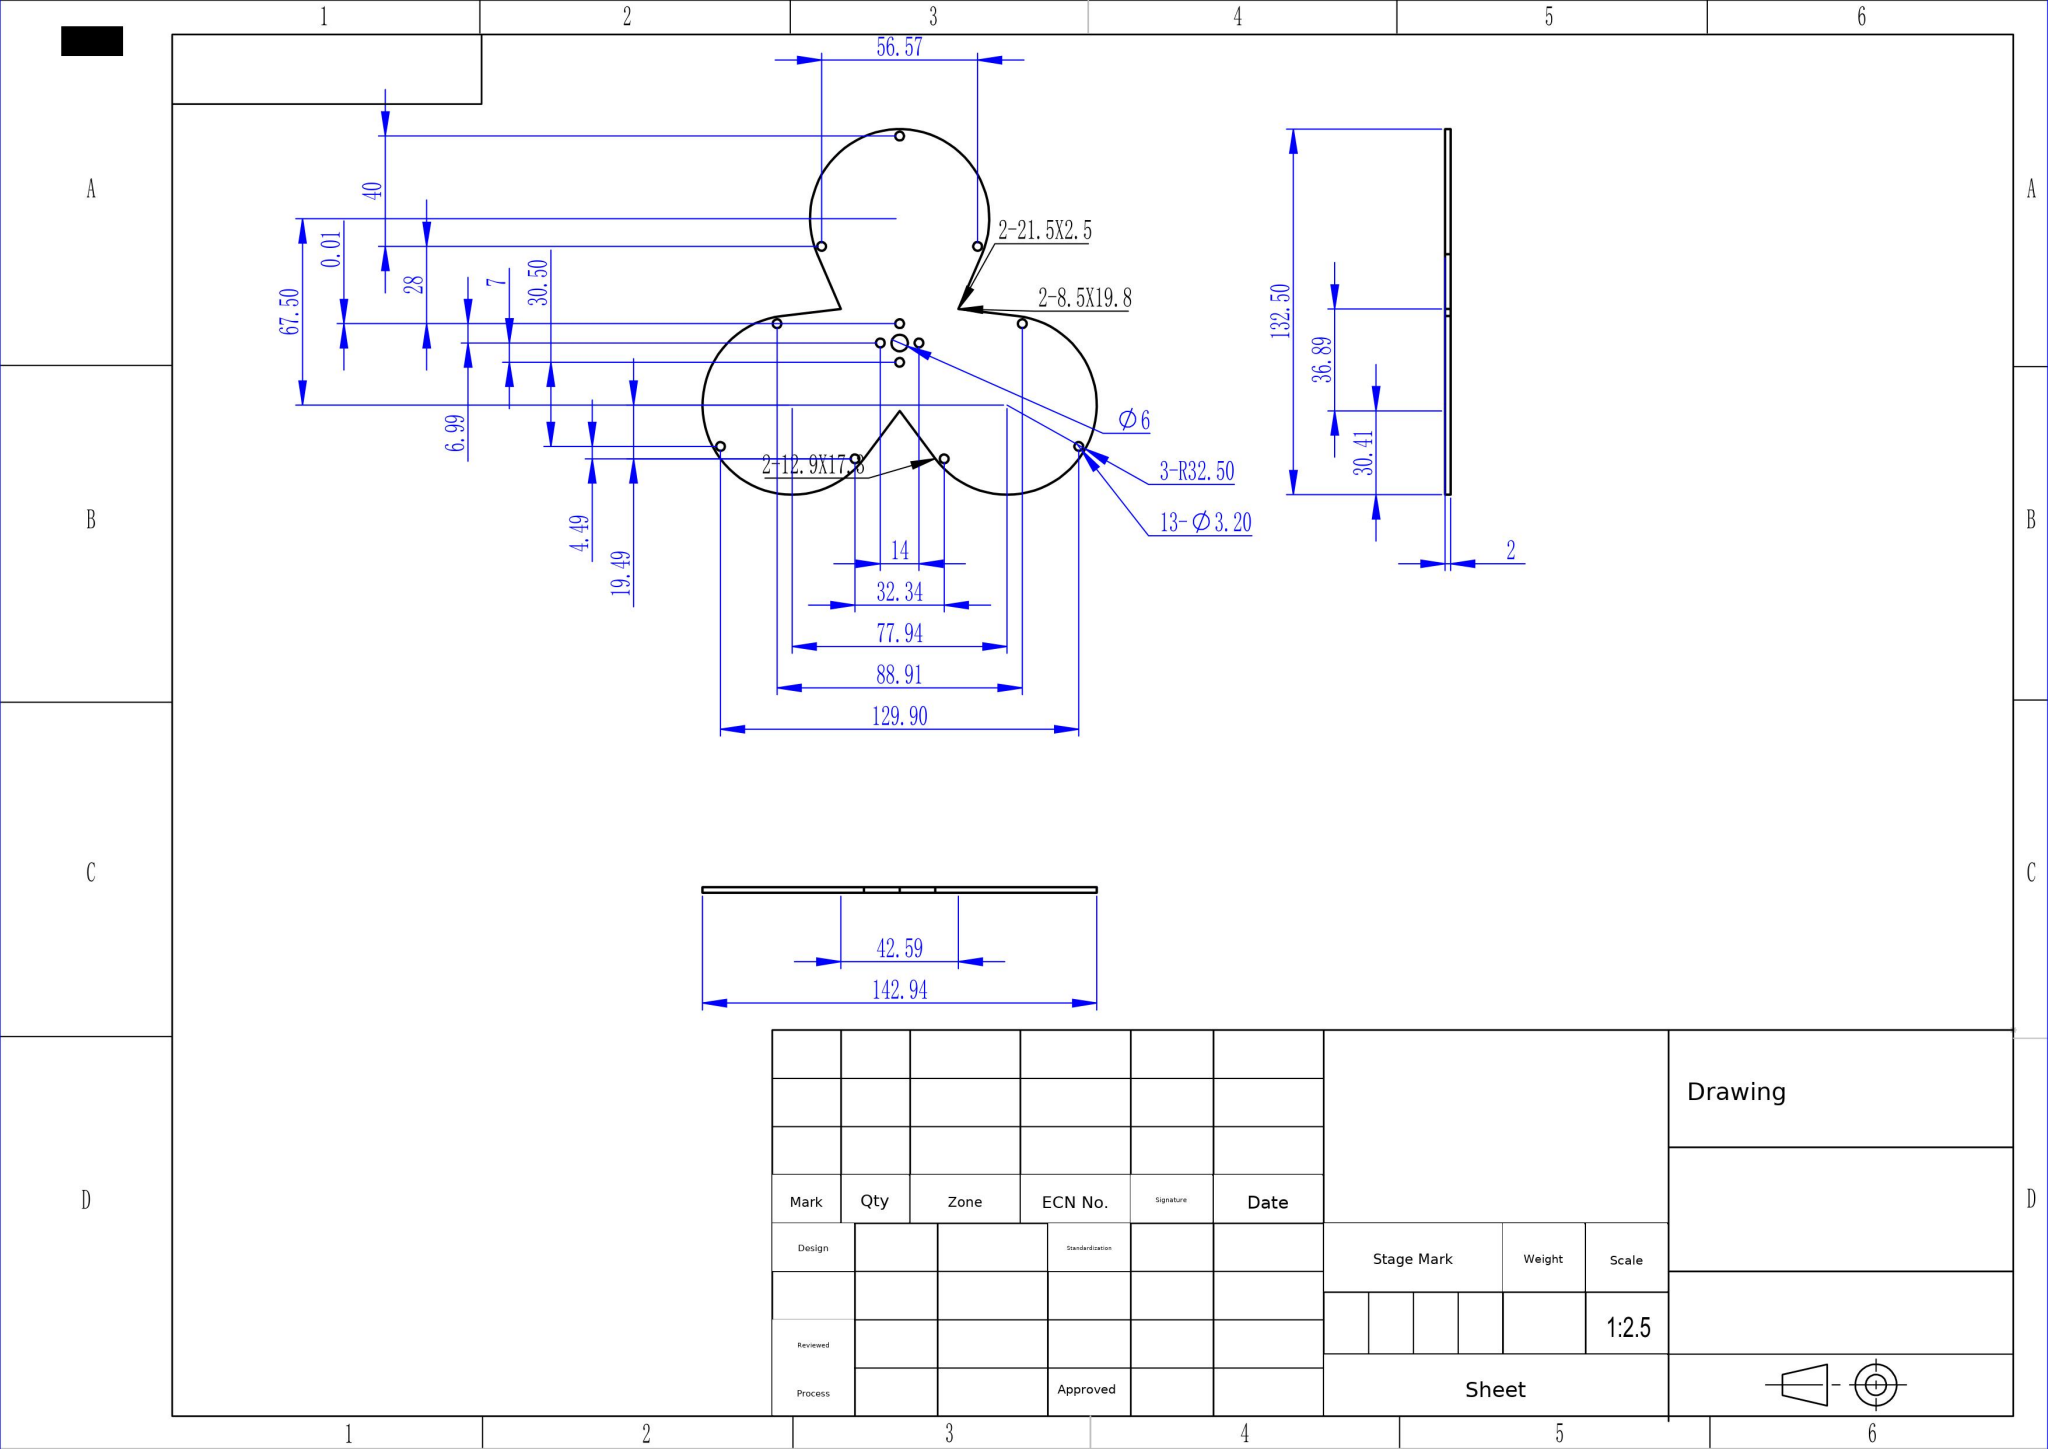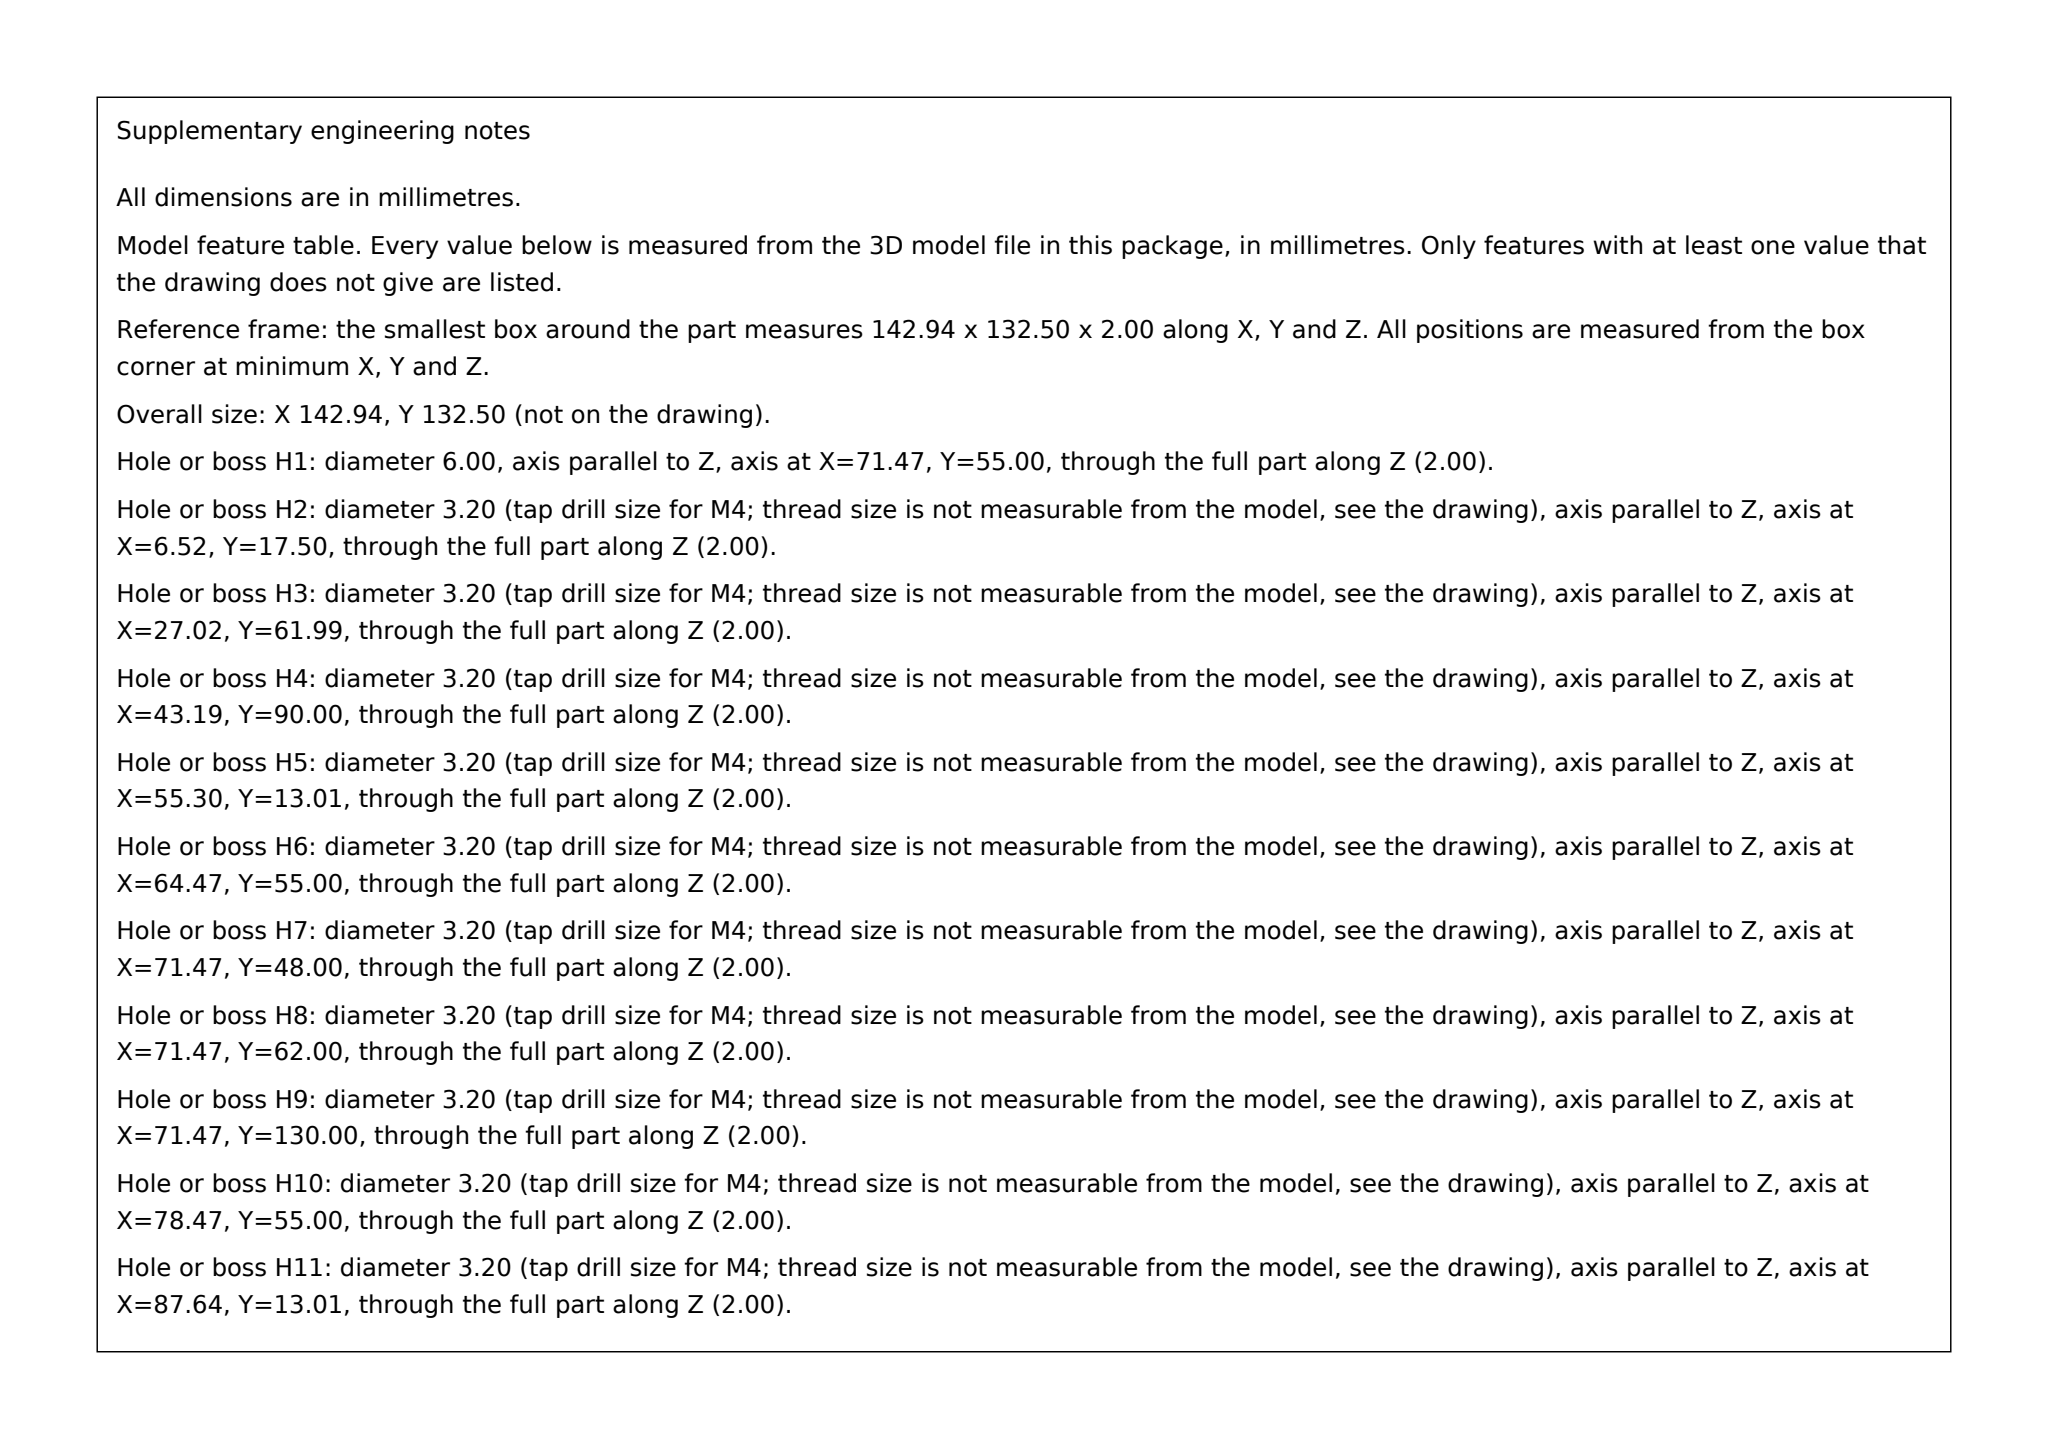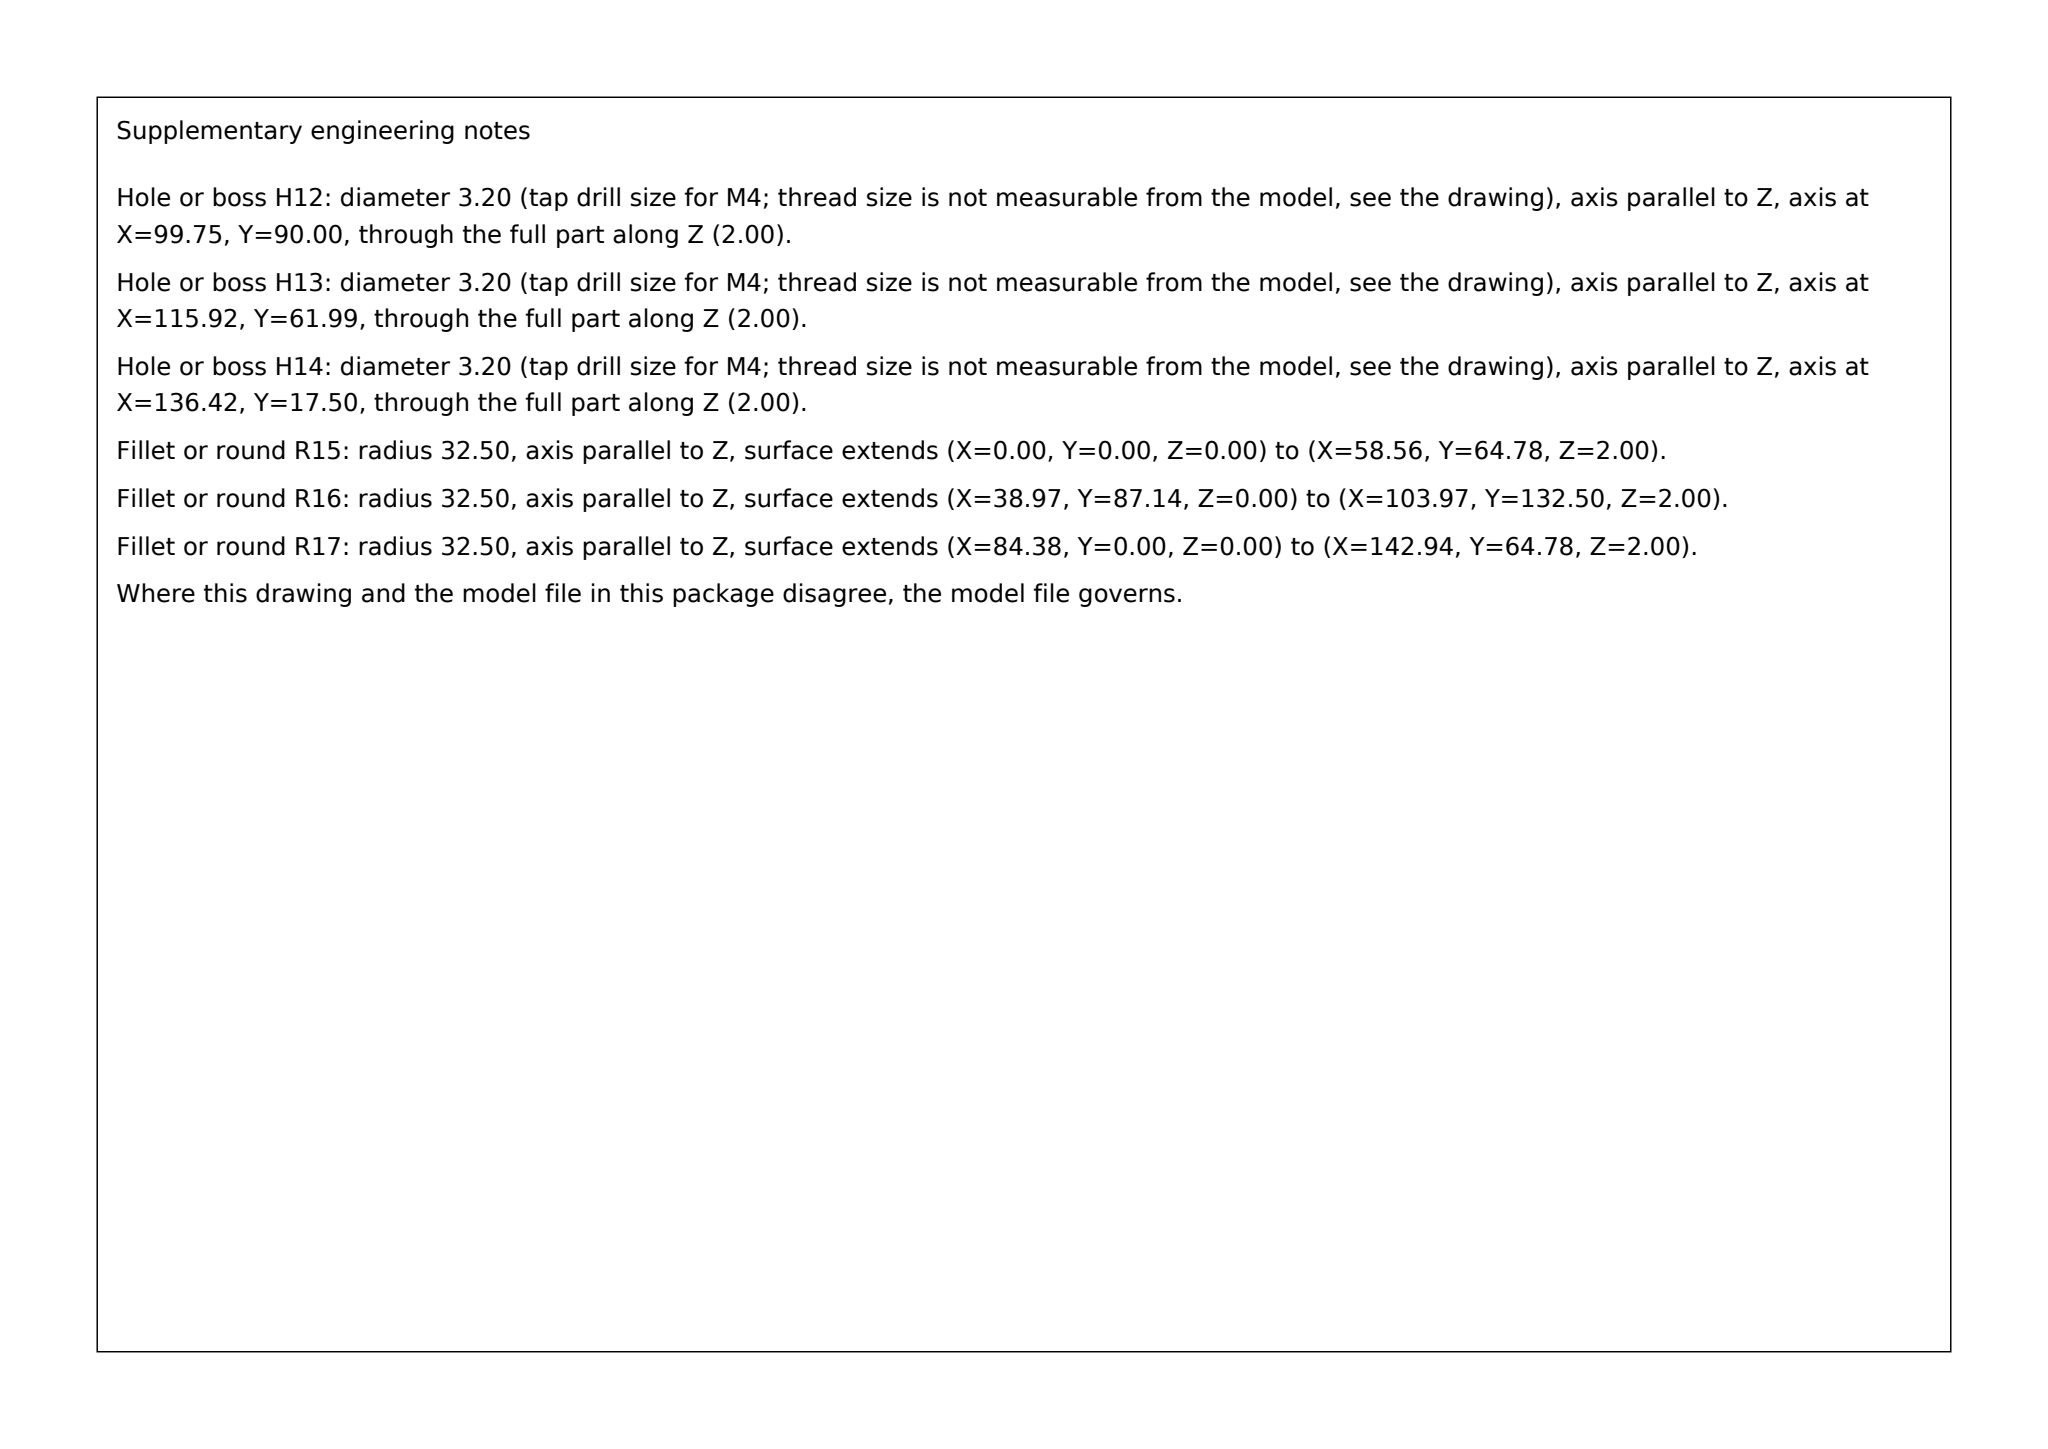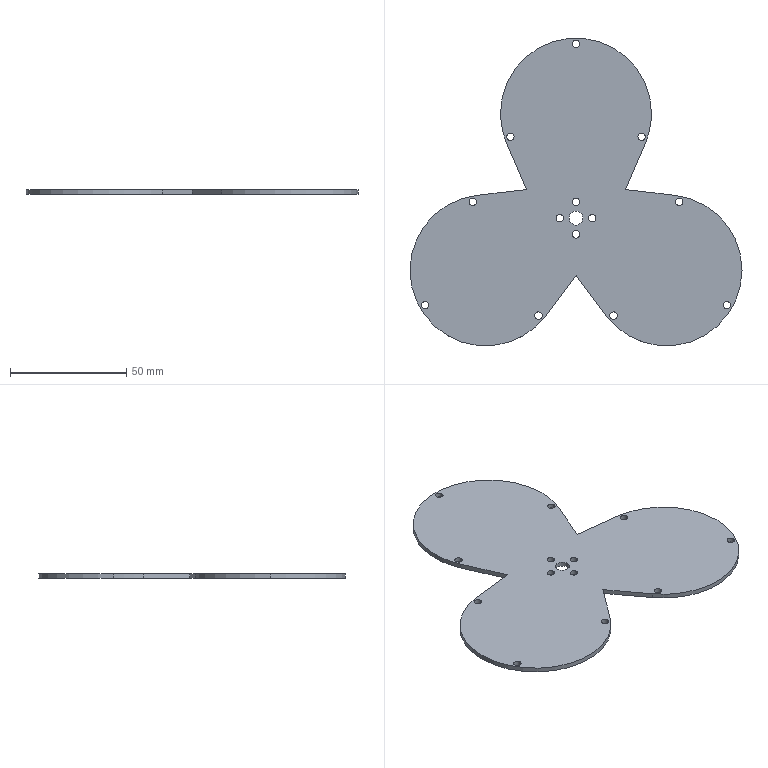Part | SolidWorks | mm | 1 solid | 42 faces | box 142.94 x 132.5 x 2 mm | volume 22231 mm3 | cylinder 34 | plane 8 | commonest cylinder face diameters 3.2 x26 65 x6 6 x2
build123d program:
from build123d import *

# Parameters (mm, degrees)
SKETCH1_R           = 1.6
SKETCH1_R_2         = 3
BOSS_EXTRUDE1_DEPTH = 2


with BuildPart() as part:
    # Sketch1 → Boss-Extrude1 (new body)
    with BuildSketch(Plane.XY):
        with BuildLine():
            Line((-29.847, 32.14), (-21.297, 12.296))
            Line((-21.297, 12.296), (-42.758, 9.779))
            ThreePointArc((-42.758, 9.779), (-67.117, -38.75), (-12.91, -41.918))
            Line((-12.91, -41.918), (0, -24.592))
            Line((0, -24.592), (12.91, -41.918))
            ThreePointArc((12.91, -41.918), (67.117, -38.75), (42.758, 9.779))
            Line((42.758, 9.779), (21.297, 12.296))
            Line((21.297, 12.296), (29.847, 32.14))
            ThreePointArc((29.847, 32.14), (0, 77.5), (-29.847, 32.14))
        make_face()
        with Locations((-7, 0)):
            Circle(SKETCH1_R, mode=Mode.SUBTRACT)
        with Locations((0, 7)):
            Circle(SKETCH1_R, mode=Mode.SUBTRACT)
        with Locations((7, 0)):
            Circle(SKETCH1_R, mode=Mode.SUBTRACT)
        with Locations((0, -7)):
            Circle(SKETCH1_R, mode=Mode.SUBTRACT)
        with Locations((-44.453, 6.995)):
            Circle(SKETCH1_R, mode=Mode.SUBTRACT)
        with Locations((-16.169, -41.995)):
            Circle(SKETCH1_R, mode=Mode.SUBTRACT)
        with Locations((-64.952, -37.5)):
            Circle(SKETCH1_R, mode=Mode.SUBTRACT)
        with Locations((44.453, 6.995)):
            Circle(SKETCH1_R, mode=Mode.SUBTRACT)
        with Locations((16.169, -41.995)):
            Circle(SKETCH1_R, mode=Mode.SUBTRACT)
        with Locations((64.952, -37.5)):
            Circle(SKETCH1_R, mode=Mode.SUBTRACT)
        with Locations((28.284, 35)):
            Circle(SKETCH1_R, mode=Mode.SUBTRACT)
        with Locations((-28.284, 35)):
            Circle(SKETCH1_R, mode=Mode.SUBTRACT)
        with Locations((0, 75)):
            Circle(SKETCH1_R, mode=Mode.SUBTRACT)
        Circle(SKETCH1_R_2, mode=Mode.SUBTRACT)
    extrude(amount=BOSS_EXTRUDE1_DEPTH)


solid = part.part